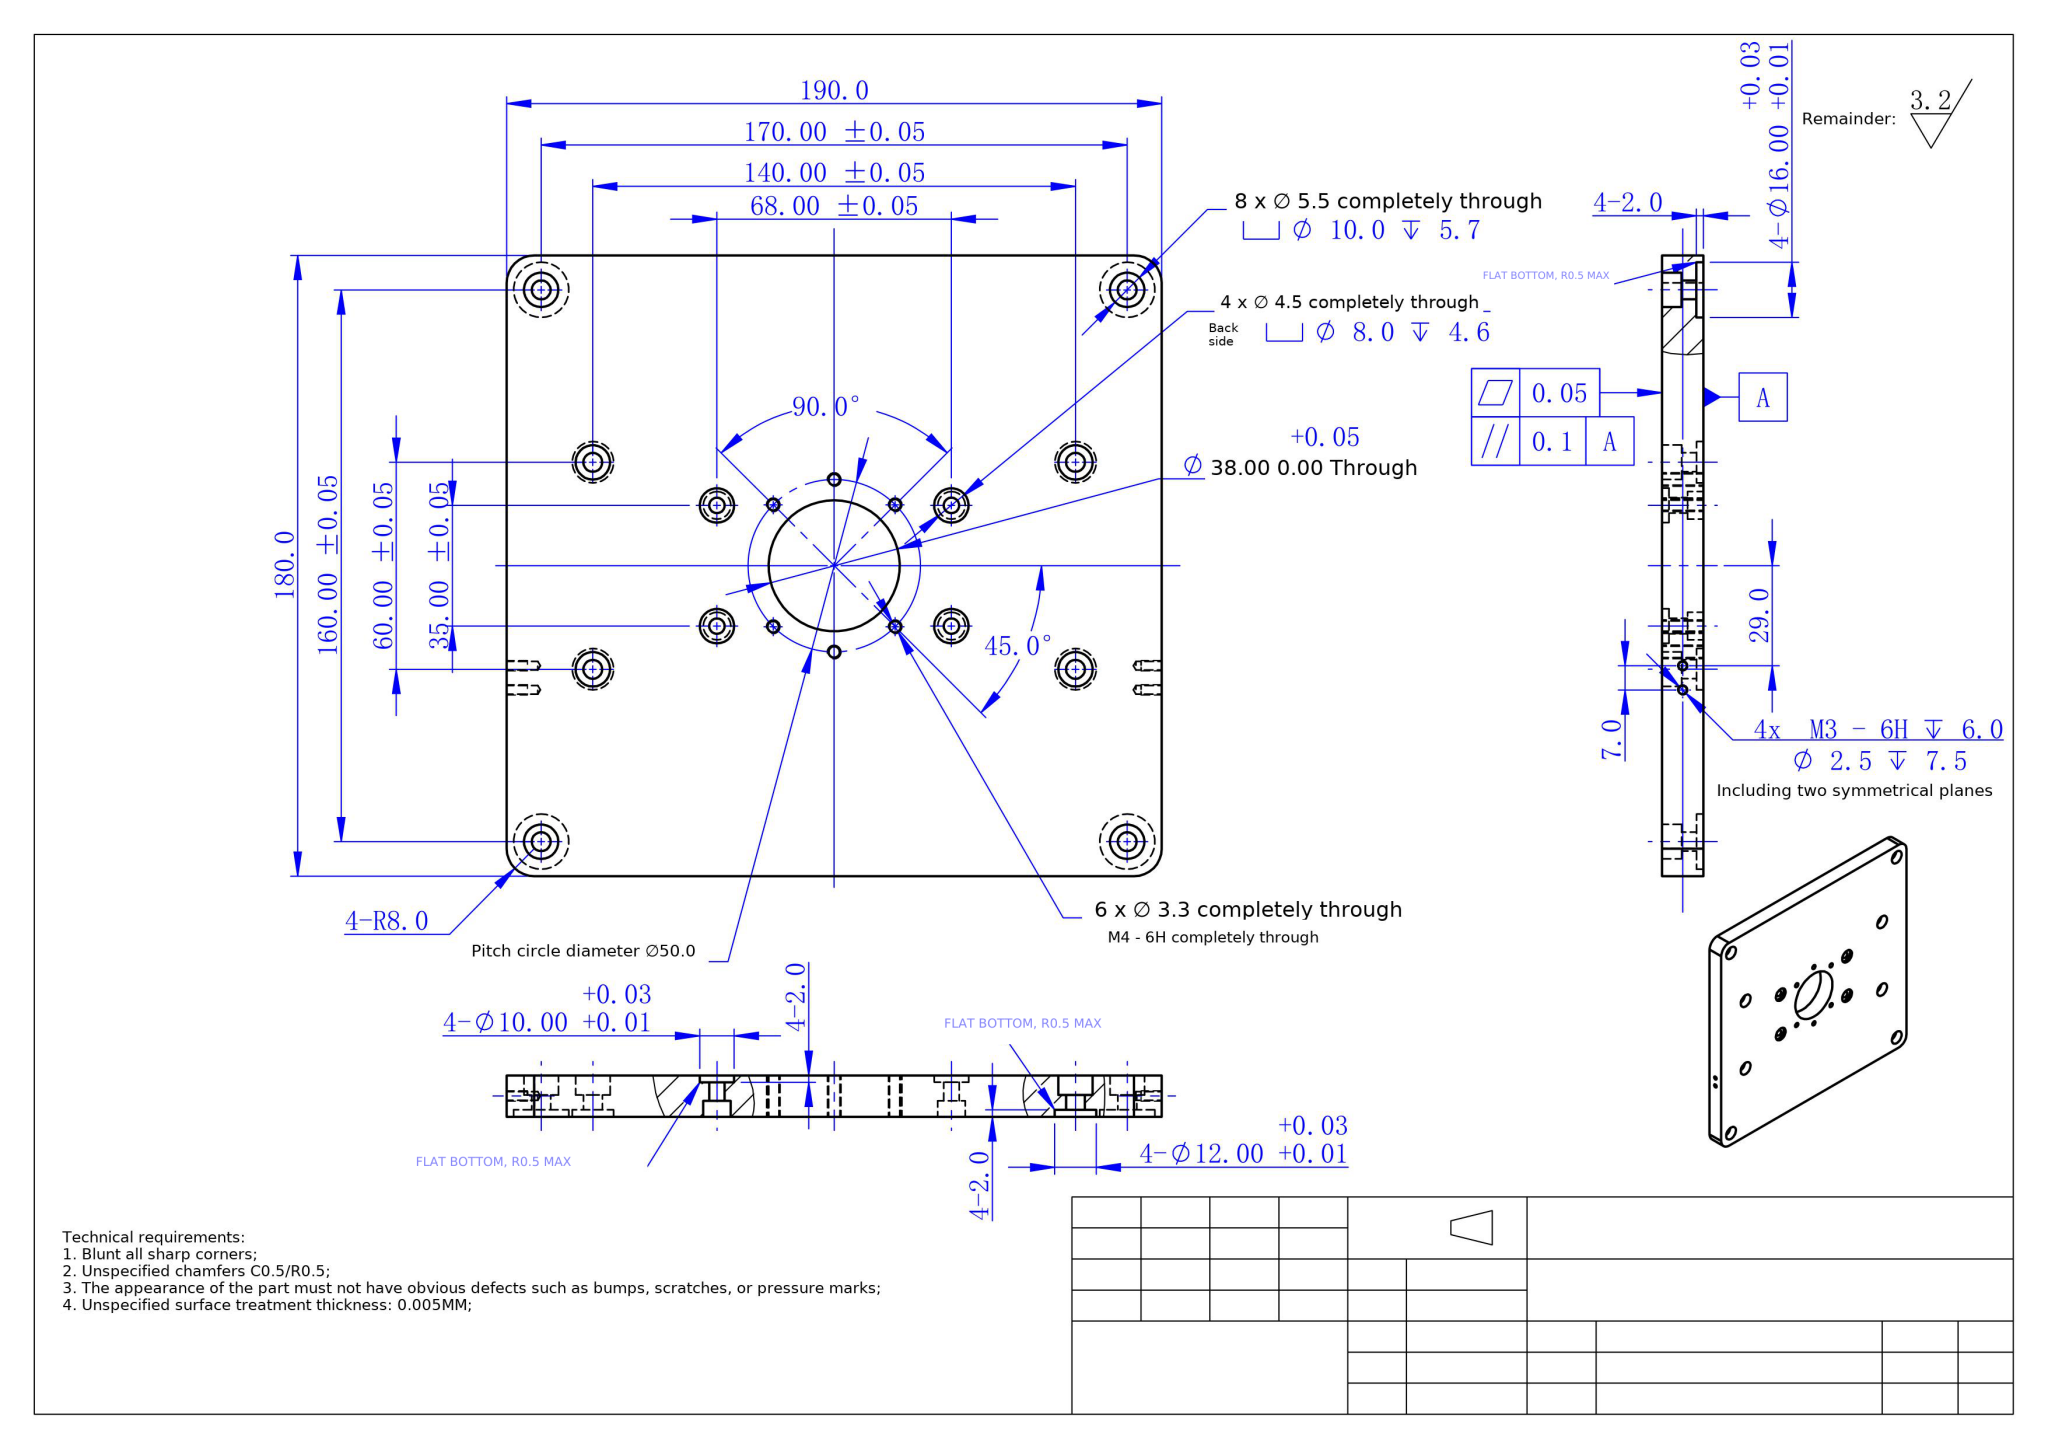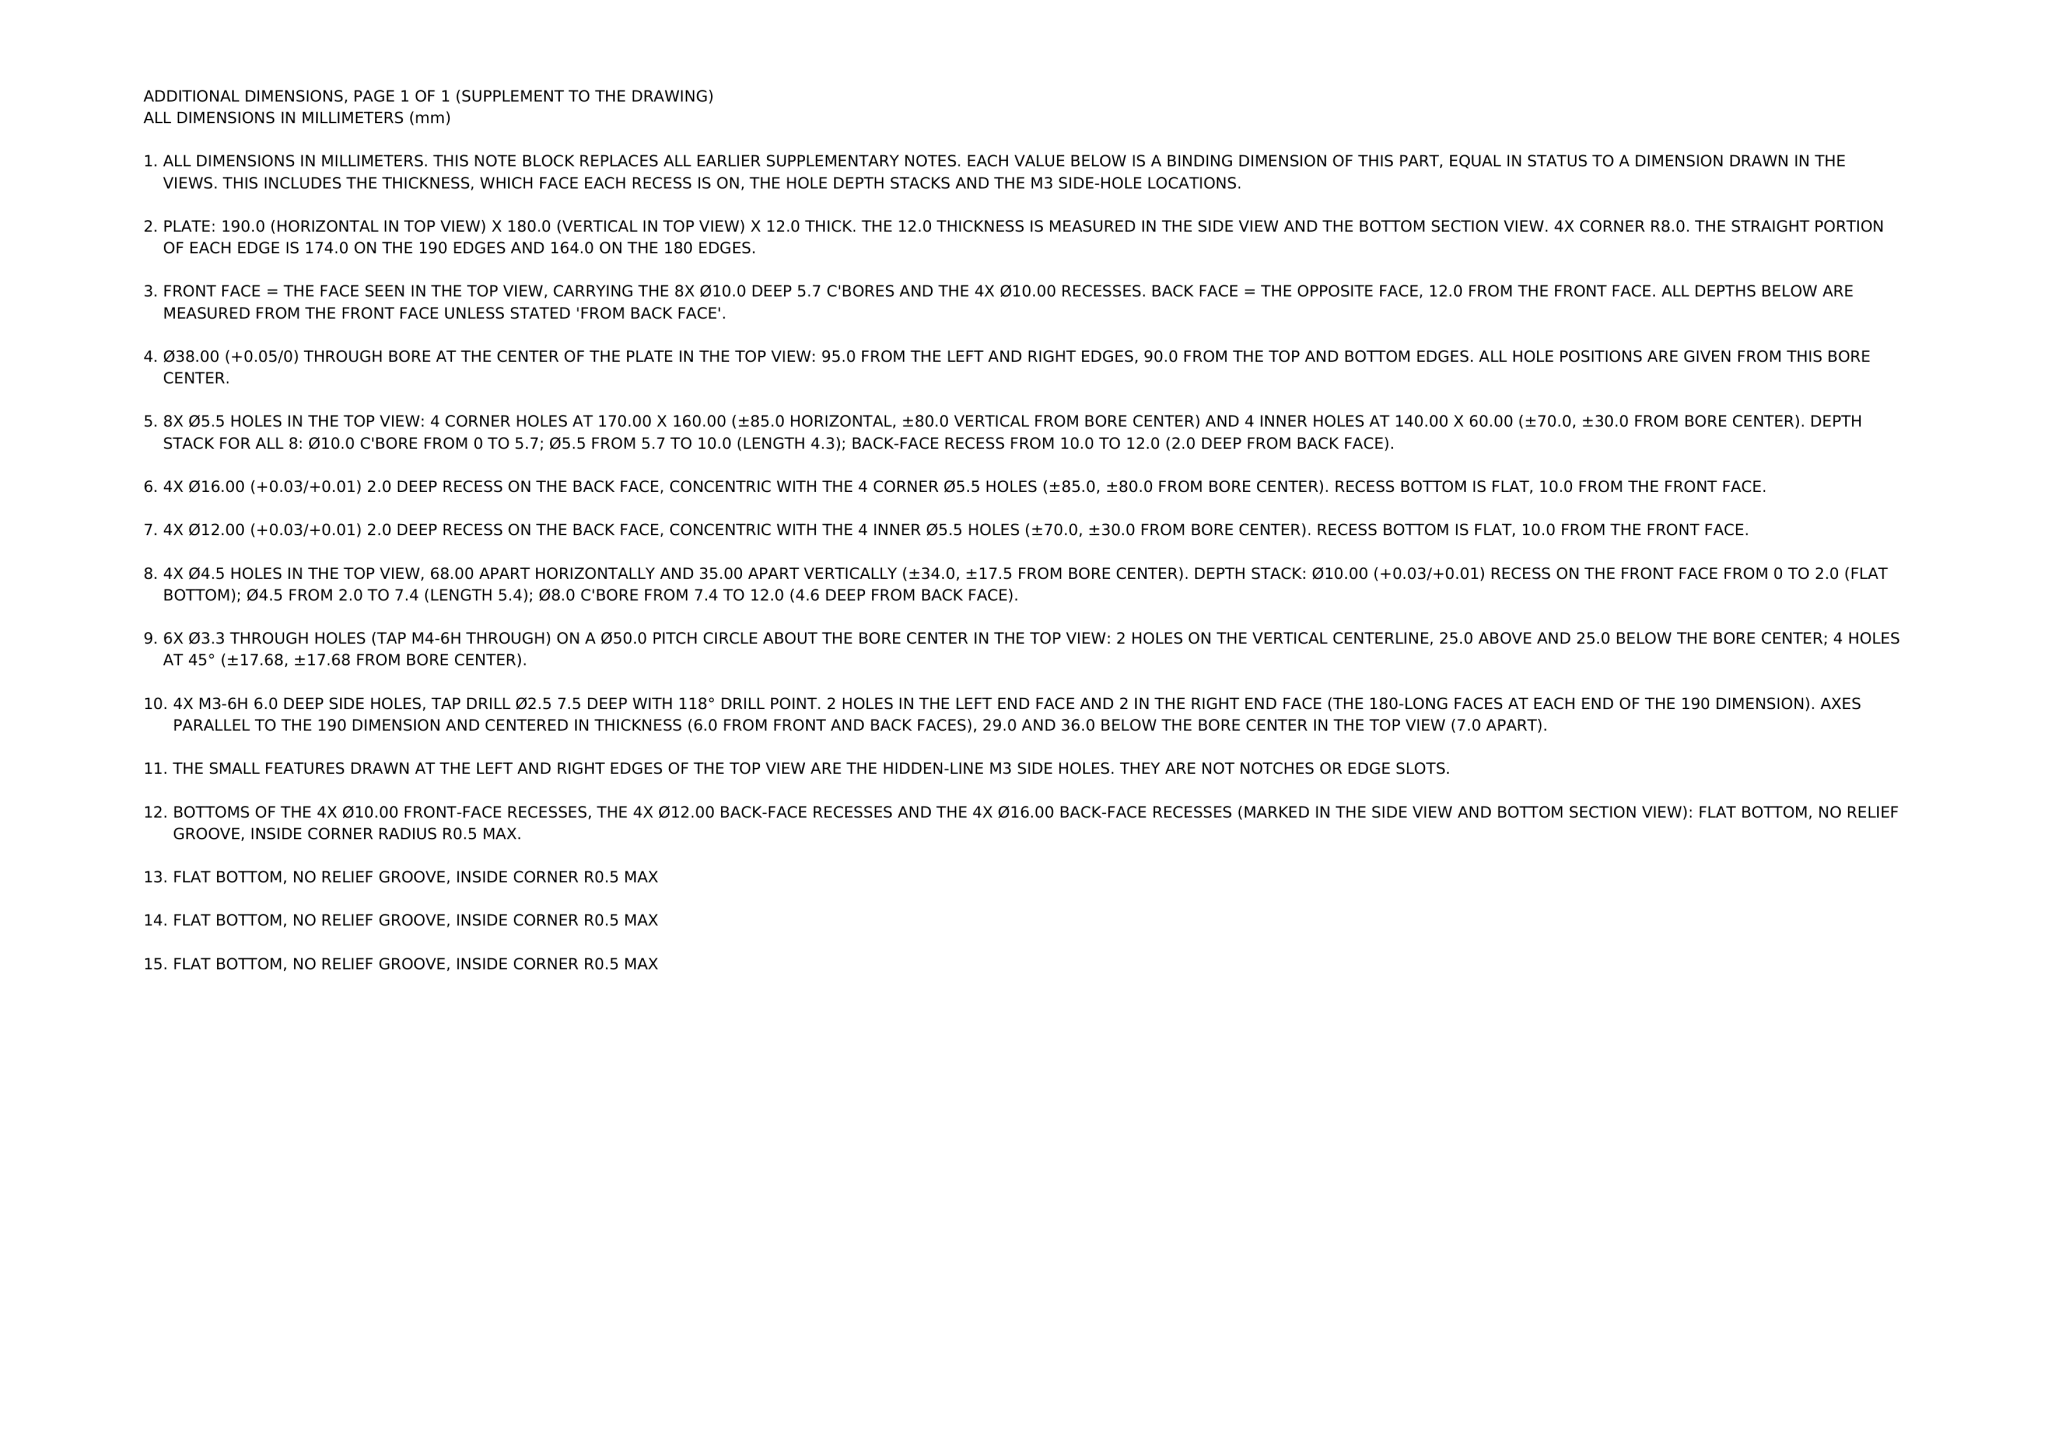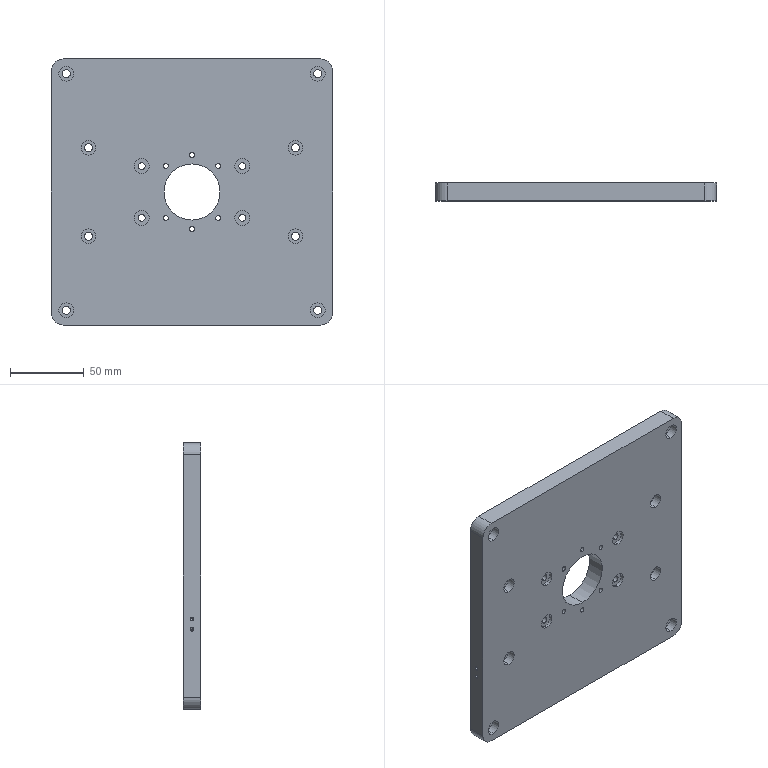Part | NX | mm | 1 solid | 136 faces | box 190 x 12 x 180 mm | volume 386540 mm3 | cylinder 98 | plane 30 | cone 8 | commonest cylinder face diameters 10 x24 5.5 x16 3.3 x12 16 x12 2.5 x8 8 x8 4.5 x8 12 x8